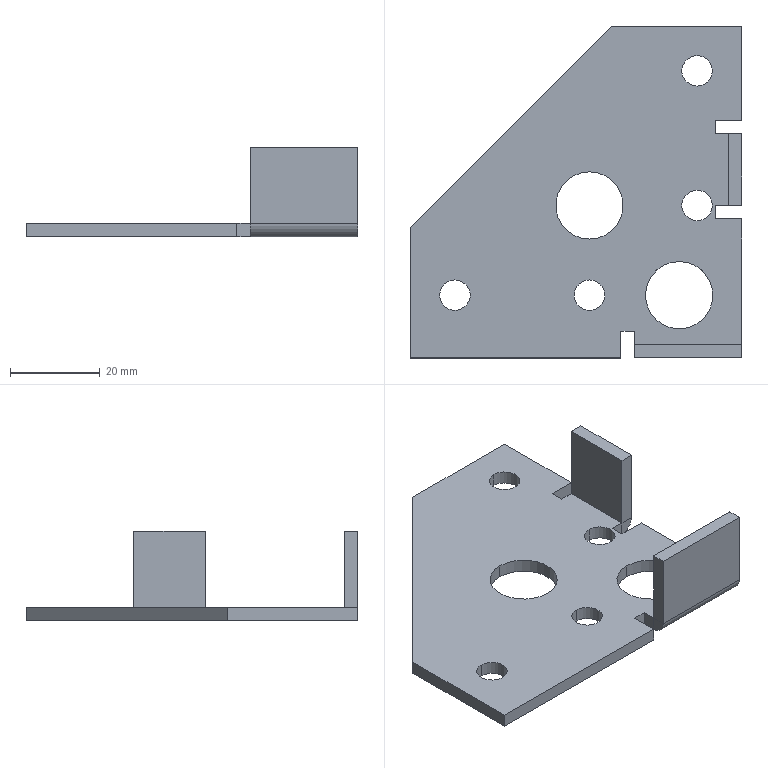Component | SolidWorks | ReinforcementPlate2-1 | 1 solid | 45 faces | volume 13695 mm3 | plane 31 | cylinder 14 | commonest cylinder face diameters 6.8 x8 15 x4 6 x2